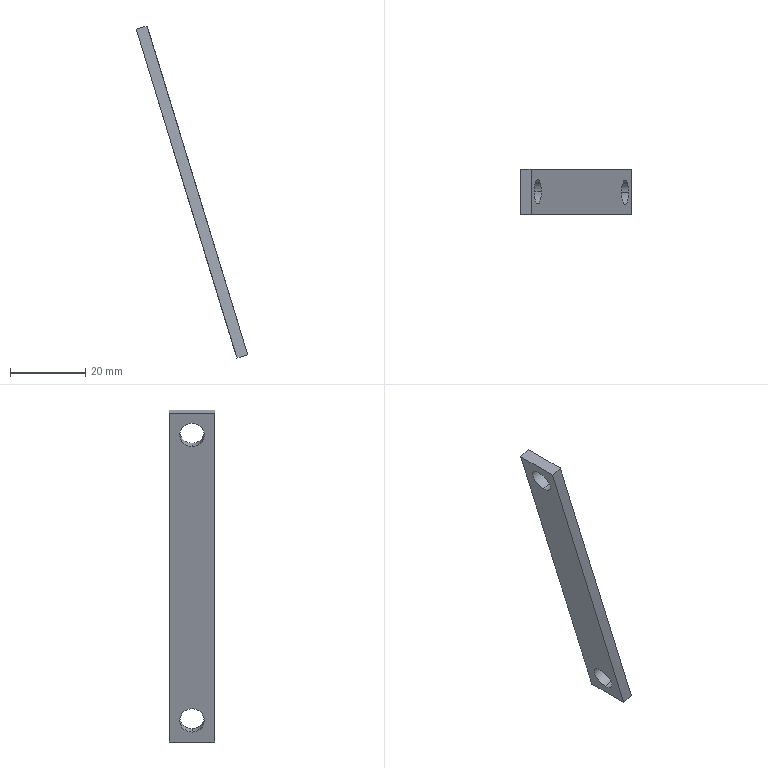Component | SolidWorks | FlatFeed-1_Part79-3 | 1 solid | 10 faces | box 29.56 x 12 x 88.19 mm | volume 3088 mm3 | plane 6 | cylinder 4 | commonest cylinder face diameters 6.5 x4
build123d program:
from build123d import *

# Parameters (mm, degrees)
SKETCH1_W          = 12
SKETCH1_H          = 91.3
EXTRUDE1_DEPTH     = 3
SKETCH2_R          = 3.25
CUT_EXTRUDE1_DEPTH = 47.14


with BuildPart() as part:
    # Sketch1 → Extrude1 (new body)
    with BuildSketch(Plane(origin=(0, 0, 0), x_dir=(1, 0, 0), z_dir=(0, 1, 0))):
        Rectangle(SKETCH1_W, SKETCH1_H)
    extrude(amount=EXTRUDE1_DEPTH)

    # Sketch2 → Cut-Extrude1 (cut, through all)
    with BuildSketch(Plane(origin=(0, 3, 0), x_dir=(1, 0, 0), z_dir=(0, 1, 0))):
        with Locations(Location((0, 39.65, 0), (0, 0, 270))):
            Circle(SKETCH2_R)
        with Locations(Location((0, -39.65, 0), (0, 0, 270))):
            Circle(SKETCH2_R)
    extrude(amount=-CUT_EXTRUDE1_DEPTH, mode=Mode.SUBTRACT)


solid = part.part

# Placed as in the assembly
solid = solid.moved(Location((121.955, -232.176, 716.655), (0, -17, 90)))
STEP:
#1=CARTESIAN_POINT('',(4.269,-9.141,29.551));
#2=VERTEX_POINT('',#1);
#3=CARTESIAN_POINT('',(4.195,-9.141,29.795));
#4=VERTEX_POINT('',#3);
#5=CARTESIAN_POINT('',(4.232,-9.141,29.673));
#6=DIRECTION('',(0.9563,0.,0.2924));
#7=DIRECTION('',(-0.2924,0.,0.9563));
#8=AXIS2_PLACEMENT_3D('',#5,#6,#7);
#9=CIRCLE('',#8,0.128);
#10=EDGE_CURVE('',#2,#4,#9,.T.);
#11=ORIENTED_EDGE('',*,*,#10,.F.);
#12=CARTESIAN_POINT('',(4.382,-9.141,29.585));
#13=VERTEX_POINT('',#12);
#14=CARTESIAN_POINT('',(4.269,-9.141,29.551));
#15=DIRECTION('',(0.9563,0.,0.2924));
#16=VECTOR('',#15,39.37);
#17=LINE('',#14,#16);
#18=EDGE_CURVE('',#2,#13,#17,.T.);
#19=ORIENTED_EDGE('',*,*,#18,.T.);
#20=CARTESIAN_POINT('',(4.308,-9.141,29.83));
#21=VERTEX_POINT('',#20);
#22=CARTESIAN_POINT('',(4.345,-9.141,29.708));
#23=DIRECTION('',(0.9563,0.,0.2924));
#24=DIRECTION('',(-0.2924,0.,0.9563));
#25=AXIS2_PLACEMENT_3D('',#22,#23,#24);
#26=CIRCLE('',#25,0.128);
#27=EDGE_CURVE('',#13,#21,#26,.T.);
#28=ORIENTED_EDGE('',*,*,#27,.T.);
#29=CARTESIAN_POINT('',(4.195,-9.141,29.795));
#30=DIRECTION('',(0.9563,0.,0.2924));
#31=VECTOR('',#30,39.37);
#32=LINE('',#29,#31);
#33=EDGE_CURVE('',#4,#21,#32,.T.);
#34=ORIENTED_EDGE('',*,*,#33,.F.);
#35=EDGE_LOOP('',(#11,#19,#28,#34));
#36=FACE_OUTER_BOUND('',#35,.T.);
#37=CARTESIAN_POINT('',(4.232,-9.141,29.673));
#38=DIRECTION('',(0.9563,0.,0.2924));
#39=DIRECTION('',(-0.2924,0.,0.9563));
#40=AXIS2_PLACEMENT_3D('',#37,#38,#39);
#41=CYLINDRICAL_SURFACE('',#40,0.128);
#42=ADVANCED_FACE('',(#36),#41,.F.);
#43=CARTESIAN_POINT('',(5.182,-9.141,26.565));
#44=VERTEX_POINT('',#43);
#45=CARTESIAN_POINT('',(5.107,-9.141,26.81));
#46=VERTEX_POINT('',#45);
#47=CARTESIAN_POINT('',(5.145,-9.141,26.687));
#48=DIRECTION('',(0.9563,0.,0.2924));
#49=DIRECTION('',(-0.2924,0.,0.9563));
#50=AXIS2_PLACEMENT_3D('',#47,#48,#49);
#51=CIRCLE('',#50,0.128);
#52=EDGE_CURVE('',#44,#46,#51,.T.);
#53=ORIENTED_EDGE('',*,*,#52,.F.);
#54=CARTESIAN_POINT('',(5.295,-9.141,26.6));
#55=VERTEX_POINT('',#54);
#56=CARTESIAN_POINT('',(5.182,-9.141,26.565));
#57=DIRECTION('',(0.9563,0.,0.2924));
#58=VECTOR('',#57,39.37);
#59=LINE('',#56,#58);
#60=EDGE_CURVE('',#44,#55,#59,.T.);
#61=ORIENTED_EDGE('',*,*,#60,.T.);
#62=CARTESIAN_POINT('',(5.22,-9.141,26.844));
#63=VERTEX_POINT('',#62);
#64=CARTESIAN_POINT('',(5.258,-9.141,26.722));
#65=DIRECTION('',(0.9563,0.,0.2924));
#66=DIRECTION('',(-0.2924,0.,0.9563));
#67=AXIS2_PLACEMENT_3D('',#64,#65,#66);
#68=CIRCLE('',#67,0.128);
#69=EDGE_CURVE('',#55,#63,#68,.T.);
#70=ORIENTED_EDGE('',*,*,#69,.T.);
#71=CARTESIAN_POINT('',(5.107,-9.141,26.81));
#72=DIRECTION('',(0.9563,0.,0.2924));
#73=VECTOR('',#72,39.37);
#74=LINE('',#71,#73);
#75=EDGE_CURVE('',#46,#63,#74,.T.);
#76=ORIENTED_EDGE('',*,*,#75,.F.);
#77=EDGE_LOOP('',(#53,#61,#70,#76));
#78=FACE_OUTER_BOUND('',#77,.T.);
#79=CARTESIAN_POINT('',(5.145,-9.141,26.687));
#80=DIRECTION('',(0.9563,0.,0.2924));
#81=DIRECTION('',(-0.2924,0.,0.9563));
#82=AXIS2_PLACEMENT_3D('',#79,#80,#81);
#83=CYLINDRICAL_SURFACE('',#82,0.128);
#84=ADVANCED_FACE('',(#78),#83,.F.);
#85=CARTESIAN_POINT('',(4.163,-9.377,29.899));
#86=VERTEX_POINT('',#85);
#87=CARTESIAN_POINT('',(5.214,-9.377,26.462));
#88=VERTEX_POINT('',#87);
#89=CARTESIAN_POINT('',(4.163,-9.377,29.899));
#90=DIRECTION('',(0.2924,-0.,-0.9563));
#91=VECTOR('',#90,39.37);
#92=LINE('',#89,#91);
#93=EDGE_CURVE('',#86,#88,#92,.T.);
#94=ORIENTED_EDGE('',*,*,#93,.T.);
#95=CARTESIAN_POINT('',(5.327,-9.377,26.496));
#96=VERTEX_POINT('',#95);
#97=CARTESIAN_POINT('',(5.327,-9.377,26.496));
#98=DIRECTION('',(-0.9563,-0.,-0.2924));
#99=VECTOR('',#98,39.37);
#100=LINE('',#97,#99);
#101=EDGE_CURVE('',#96,#88,#100,.T.);
#102=ORIENTED_EDGE('',*,*,#101,.F.);
#103=CARTESIAN_POINT('',(4.276,-9.377,29.933));
#104=VERTEX_POINT('',#103);
#105=CARTESIAN_POINT('',(4.276,-9.377,29.933));
#106=DIRECTION('',(0.2924,-0.,-0.9563));
#107=VECTOR('',#106,39.37);
#108=LINE('',#105,#107);
#109=EDGE_CURVE('',#104,#96,#108,.T.);
#110=ORIENTED_EDGE('',*,*,#109,.F.);
#111=CARTESIAN_POINT('',(4.276,-9.377,29.933));
#112=DIRECTION('',(-0.9563,-0.,-0.2924));
#113=VECTOR('',#112,39.37);
#114=LINE('',#111,#113);
#115=EDGE_CURVE('',#104,#86,#114,.T.);
#116=ORIENTED_EDGE('',*,*,#115,.T.);
#117=EDGE_LOOP('',(#94,#102,#110,#116));
#118=FACE_OUTER_BOUND('',#117,.T.);
#119=CARTESIAN_POINT('',(4.276,-9.377,29.933));
#120=DIRECTION('',(-0.,1.,-0.));
#121=DIRECTION('',(-0.2924,0.,0.9563));
#122=AXIS2_PLACEMENT_3D('',#119,#120,#121);
#123=PLANE('',#122);
#124=ADVANCED_FACE('',(#118),#123,.F.);
#125=CARTESIAN_POINT('',(5.214,-8.905,26.462));
#126=VERTEX_POINT('',#125);
#127=CARTESIAN_POINT('',(5.214,-8.905,26.462));
#128=DIRECTION('',(-0.,1.,-0.));
#129=VECTOR('',#128,39.37);
#130=LINE('',#127,#129);
#131=EDGE_CURVE('',#88,#126,#130,.T.);
#132=ORIENTED_EDGE('',*,*,#131,.T.);
#133=CARTESIAN_POINT('',(5.327,-8.905,26.496));
#134=VERTEX_POINT('',#133);
#135=CARTESIAN_POINT('',(5.327,-8.905,26.496));
#136=DIRECTION('',(-0.9563,-0.,-0.2924));
#137=VECTOR('',#136,39.37);
#138=LINE('',#135,#137);
#139=EDGE_CURVE('',#134,#126,#138,.T.);
#140=ORIENTED_EDGE('',*,*,#139,.F.);
#141=CARTESIAN_POINT('',(5.327,-8.905,26.496));
#142=DIRECTION('',(-0.,1.,-0.));
#143=VECTOR('',#142,39.37);
#144=LINE('',#141,#143);
#145=EDGE_CURVE('',#96,#134,#144,.T.);
#146=ORIENTED_EDGE('',*,*,#145,.F.);
#147=ORIENTED_EDGE('',*,*,#101,.T.);
#148=EDGE_LOOP('',(#132,#140,#146,#147));
#149=FACE_OUTER_BOUND('',#148,.T.);
#150=CARTESIAN_POINT('',(5.327,-8.905,26.496));
#151=DIRECTION('',(-0.2924,0.,0.9563));
#152=DIRECTION('',(0.,-1.,0.));
#153=AXIS2_PLACEMENT_3D('',#150,#151,#152);
#154=PLANE('',#153);
#155=ADVANCED_FACE('',(#149),#154,.F.);
#156=CARTESIAN_POINT('',(4.163,-8.905,29.899));
#157=VERTEX_POINT('',#156);
#158=CARTESIAN_POINT('',(4.163,-8.905,29.899));
#159=DIRECTION('',(-0.2924,0.,0.9563));
#160=VECTOR('',#159,39.37);
#161=LINE('',#158,#160);
#162=EDGE_CURVE('',#126,#157,#161,.T.);
#163=ORIENTED_EDGE('',*,*,#162,.T.);
#164=CARTESIAN_POINT('',(4.276,-8.905,29.933));
#165=VERTEX_POINT('',#164);
#166=CARTESIAN_POINT('',(4.276,-8.905,29.933));
#167=DIRECTION('',(-0.9563,-0.,-0.2924));
#168=VECTOR('',#167,39.37);
#169=LINE('',#166,#168);
#170=EDGE_CURVE('',#165,#157,#169,.T.);
#171=ORIENTED_EDGE('',*,*,#170,.F.);
#172=CARTESIAN_POINT('',(4.276,-8.905,29.933));
#173=DIRECTION('',(-0.2924,0.,0.9563));
#174=VECTOR('',#173,39.37);
#175=LINE('',#172,#174);
#176=EDGE_CURVE('',#134,#165,#175,.T.);
#177=ORIENTED_EDGE('',*,*,#176,.F.);
#178=ORIENTED_EDGE('',*,*,#139,.T.);
#179=EDGE_LOOP('',(#163,#171,#177,#178));
#180=FACE_OUTER_BOUND('',#179,.T.);
#181=CARTESIAN_POINT('',(4.276,-8.905,29.933));
#182=DIRECTION('',(0.,-1.,0.));
#183=DIRECTION('',(0.2924,-0.,-0.9563));
#184=AXIS2_PLACEMENT_3D('',#181,#182,#183);
#185=PLANE('',#184);
#186=ADVANCED_FACE('',(#180),#185,.F.);
#187=CARTESIAN_POINT('',(4.163,-8.905,29.899));
#188=DIRECTION('',(0.,-1.,0.));
#189=VECTOR('',#188,39.37);
#190=LINE('',#187,#189);
#191=EDGE_CURVE('',#157,#86,#190,.T.);
#192=ORIENTED_EDGE('',*,*,#191,.T.);
#193=ORIENTED_EDGE('',*,*,#115,.F.);
#194=CARTESIAN_POINT('',(4.276,-8.905,29.933));
#195=DIRECTION('',(0.,-1.,0.));
#196=VECTOR('',#195,39.37);
#197=LINE('',#194,#196);
#198=EDGE_CURVE('',#165,#104,#197,.T.);
#199=ORIENTED_EDGE('',*,*,#198,.F.);
#200=ORIENTED_EDGE('',*,*,#170,.T.);
#201=EDGE_LOOP('',(#192,#193,#199,#200));
#202=FACE_OUTER_BOUND('',#201,.T.);
#203=CARTESIAN_POINT('',(4.276,-8.905,29.933));
#204=DIRECTION('',(0.2924,-0.,-0.9563));
#205=DIRECTION('',(-0.,1.,-0.));
#206=AXIS2_PLACEMENT_3D('',#203,#204,#205);
#207=PLANE('',#206);
#208=ADVANCED_FACE('',(#202),#207,.F.);
#209=CARTESIAN_POINT('',(4.345,-9.141,29.708));
#210=DIRECTION('',(0.9563,0.,0.2924));
#211=DIRECTION('',(-0.2924,0.,0.9563));
#212=AXIS2_PLACEMENT_3D('',#209,#210,#211);
#213=CIRCLE('',#212,0.128);
#214=EDGE_CURVE('',#21,#13,#213,.T.);
#215=ORIENTED_EDGE('',*,*,#214,.F.);
#216=ORIENTED_EDGE('',*,*,#27,.F.);
#217=EDGE_LOOP('',(#215,#216));
#218=FACE_BOUND('',#217,.T.);
#219=CARTESIAN_POINT('',(5.258,-9.141,26.722));
#220=DIRECTION('',(0.9563,0.,0.2924));
#221=DIRECTION('',(-0.2924,0.,0.9563));
#222=AXIS2_PLACEMENT_3D('',#219,#220,#221);
#223=CIRCLE('',#222,0.128);
#224=EDGE_CURVE('',#63,#55,#223,.T.);
#225=ORIENTED_EDGE('',*,*,#224,.F.);
#226=ORIENTED_EDGE('',*,*,#69,.F.);
#227=EDGE_LOOP('',(#225,#226));
#228=FACE_BOUND('',#227,.T.);
#229=ORIENTED_EDGE('',*,*,#109,.T.);
#230=ORIENTED_EDGE('',*,*,#145,.T.);
#231=ORIENTED_EDGE('',*,*,#176,.T.);
#232=ORIENTED_EDGE('',*,*,#198,.T.);
#233=EDGE_LOOP('',(#229,#230,#231,#232));
#234=FACE_OUTER_BOUND('',#233,.T.);
#235=CARTESIAN_POINT('',(5.327,-9.377,26.496));
#236=DIRECTION('',(-0.9563,-0.,-0.2924));
#237=DIRECTION('',(0.2924,-0.,-0.9563));
#238=AXIS2_PLACEMENT_3D('',#235,#236,#237);
#239=PLANE('',#238);
#240=ADVANCED_FACE('',(#218,#228,#234),#239,.F.);
#241=CARTESIAN_POINT('',(4.232,-9.141,29.673));
#242=DIRECTION('',(0.9563,0.,0.2924));
#243=DIRECTION('',(-0.2924,0.,0.9563));
#244=AXIS2_PLACEMENT_3D('',#241,#242,#243);
#245=CIRCLE('',#244,0.128);
#246=EDGE_CURVE('',#4,#2,#245,.T.);
#247=ORIENTED_EDGE('',*,*,#246,.T.);
#248=ORIENTED_EDGE('',*,*,#10,.T.);
#249=EDGE_LOOP('',(#247,#248));
#250=FACE_BOUND('',#249,.T.);
#251=CARTESIAN_POINT('',(5.145,-9.141,26.687));
#252=DIRECTION('',(0.9563,0.,0.2924));
#253=DIRECTION('',(-0.2924,0.,0.9563));
#254=AXIS2_PLACEMENT_3D('',#251,#252,#253);
#255=CIRCLE('',#254,0.128);
#256=EDGE_CURVE('',#46,#44,#255,.T.);
#257=ORIENTED_EDGE('',*,*,#256,.T.);
#258=ORIENTED_EDGE('',*,*,#52,.T.);
#259=EDGE_LOOP('',(#257,#258));
#260=FACE_BOUND('',#259,.T.);
#261=ORIENTED_EDGE('',*,*,#93,.F.);
#262=ORIENTED_EDGE('',*,*,#191,.F.);
#263=ORIENTED_EDGE('',*,*,#162,.F.);
#264=ORIENTED_EDGE('',*,*,#131,.F.);
#265=EDGE_LOOP('',(#261,#262,#263,#264));
#266=FACE_OUTER_BOUND('',#265,.T.);
#267=CARTESIAN_POINT('',(5.214,-9.377,26.462));
#268=DIRECTION('',(-0.9563,-0.,-0.2924));
#269=DIRECTION('',(0.2924,-0.,-0.9563));
#270=AXIS2_PLACEMENT_3D('',#267,#268,#269);
#271=PLANE('',#270);
#272=ADVANCED_FACE('',(#250,#260,#266),#271,.T.);
#273=ORIENTED_EDGE('',*,*,#60,.F.);
#274=ORIENTED_EDGE('',*,*,#256,.F.);
#275=ORIENTED_EDGE('',*,*,#75,.T.);
#276=ORIENTED_EDGE('',*,*,#224,.T.);
#277=EDGE_LOOP('',(#273,#274,#275,#276));
#278=FACE_OUTER_BOUND('',#277,.T.);
#279=CARTESIAN_POINT('',(5.145,-9.141,26.687));
#280=DIRECTION('',(0.9563,0.,0.2924));
#281=DIRECTION('',(-0.2924,0.,0.9563));
#282=AXIS2_PLACEMENT_3D('',#279,#280,#281);
#283=CYLINDRICAL_SURFACE('',#282,0.128);
#284=ADVANCED_FACE('',(#278),#283,.F.);
#285=ORIENTED_EDGE('',*,*,#18,.F.);
#286=ORIENTED_EDGE('',*,*,#246,.F.);
#287=ORIENTED_EDGE('',*,*,#33,.T.);
#288=ORIENTED_EDGE('',*,*,#214,.T.);
#289=EDGE_LOOP('',(#285,#286,#287,#288));
#290=FACE_OUTER_BOUND('',#289,.T.);
#291=CARTESIAN_POINT('',(4.232,-9.141,29.673));
#292=DIRECTION('',(0.9563,0.,0.2924));
#293=DIRECTION('',(-0.2924,0.,0.9563));
#294=AXIS2_PLACEMENT_3D('',#291,#292,#293);
#295=CYLINDRICAL_SURFACE('',#294,0.128);
#296=ADVANCED_FACE('',(#290),#295,.F.);
#297=CLOSED_SHELL('',(#42,#84,#124,#155,#186,#208,#240,#272,#284,#296));
#298=MANIFOLD_SOLID_BREP('',#297);
#299=CARTESIAN_POINT('',(0.,0.,0.));
#300=DIRECTION('',(0.,0.,1.));
#301=DIRECTION('',(1.,0.,0.));
#302=AXIS2_PLACEMENT_3D('',#299,#300,#301);
#303=(LENGTH_UNIT()NAMED_UNIT(*)SI_UNIT($,.METRE.));
#304=LENGTH_MEASURE_WITH_UNIT(LENGTH_MEASURE(0.0254),#303);
#305=DIMENSIONAL_EXPONENTS(1.,0.,0.,0.,0.,0.,0.);
#306=(CONVERSION_BASED_UNIT('',#304)LENGTH_UNIT()NAMED_UNIT(#305));
#307=UNCERTAINTY_MEASURE_WITH_UNIT(LENGTH_MEASURE(0.00001),#306,'','');
#308=(NAMED_UNIT(*)PLANE_ANGLE_UNIT()SI_UNIT($,.RADIAN.));
#309=(NAMED_UNIT(*)SI_UNIT($,.STERADIAN.)SOLID_ANGLE_UNIT());
#310=(GEOMETRIC_REPRESENTATION_CONTEXT(3)GLOBAL_UNCERTAINTY_ASSIGNED_CONTEXT((#307))GLOBAL_UNIT_ASSIGNED_CONTEXT((#306,#308,#309))REPRESENTATION_CONTEXT('',''));
#311=ADVANCED_BREP_SHAPE_REPRESENTATION('',(#298,#302),#310);
#312=COLOUR_RGB('',0.7922,0.8196,0.9333);
#313=FILL_AREA_STYLE_COLOUR('',#312);
#314=FILL_AREA_STYLE('',(#313));
#315=SURFACE_STYLE_FILL_AREA(#314);
#316=SURFACE_SIDE_STYLE('',(#315));
#317=SURFACE_STYLE_USAGE(.BOTH.,#316);
#318=PRESENTATION_STYLE_ASSIGNMENT((#317));
#319=STYLED_ITEM('',(#318),#298);
#320=(LENGTH_UNIT()NAMED_UNIT(*)SI_UNIT($,.METRE.));
#321=LENGTH_MEASURE_WITH_UNIT(LENGTH_MEASURE(0.0254),#320);
#322=DIMENSIONAL_EXPONENTS(1.,0.,0.,0.,0.,0.,0.);
#323=(CONVERSION_BASED_UNIT('',#321)LENGTH_UNIT()NAMED_UNIT(#322));
#324=UNCERTAINTY_MEASURE_WITH_UNIT(LENGTH_MEASURE(0.00001),#323,'','');
#325=(NAMED_UNIT(*)PLANE_ANGLE_UNIT()SI_UNIT($,.RADIAN.));
#326=(NAMED_UNIT(*)SI_UNIT($,.STERADIAN.)SOLID_ANGLE_UNIT());
#327=(GEOMETRIC_REPRESENTATION_CONTEXT(3)GLOBAL_UNCERTAINTY_ASSIGNED_CONTEXT((#324))GLOBAL_UNIT_ASSIGNED_CONTEXT((#323,#325,#326))REPRESENTATION_CONTEXT('',''));
#328=MECHANICAL_DESIGN_GEOMETRIC_PRESENTATION_REPRESENTATION('',(#319),#327);
#329=PRESENTATION_LAYER_ASSIGNMENT('','',(#319));